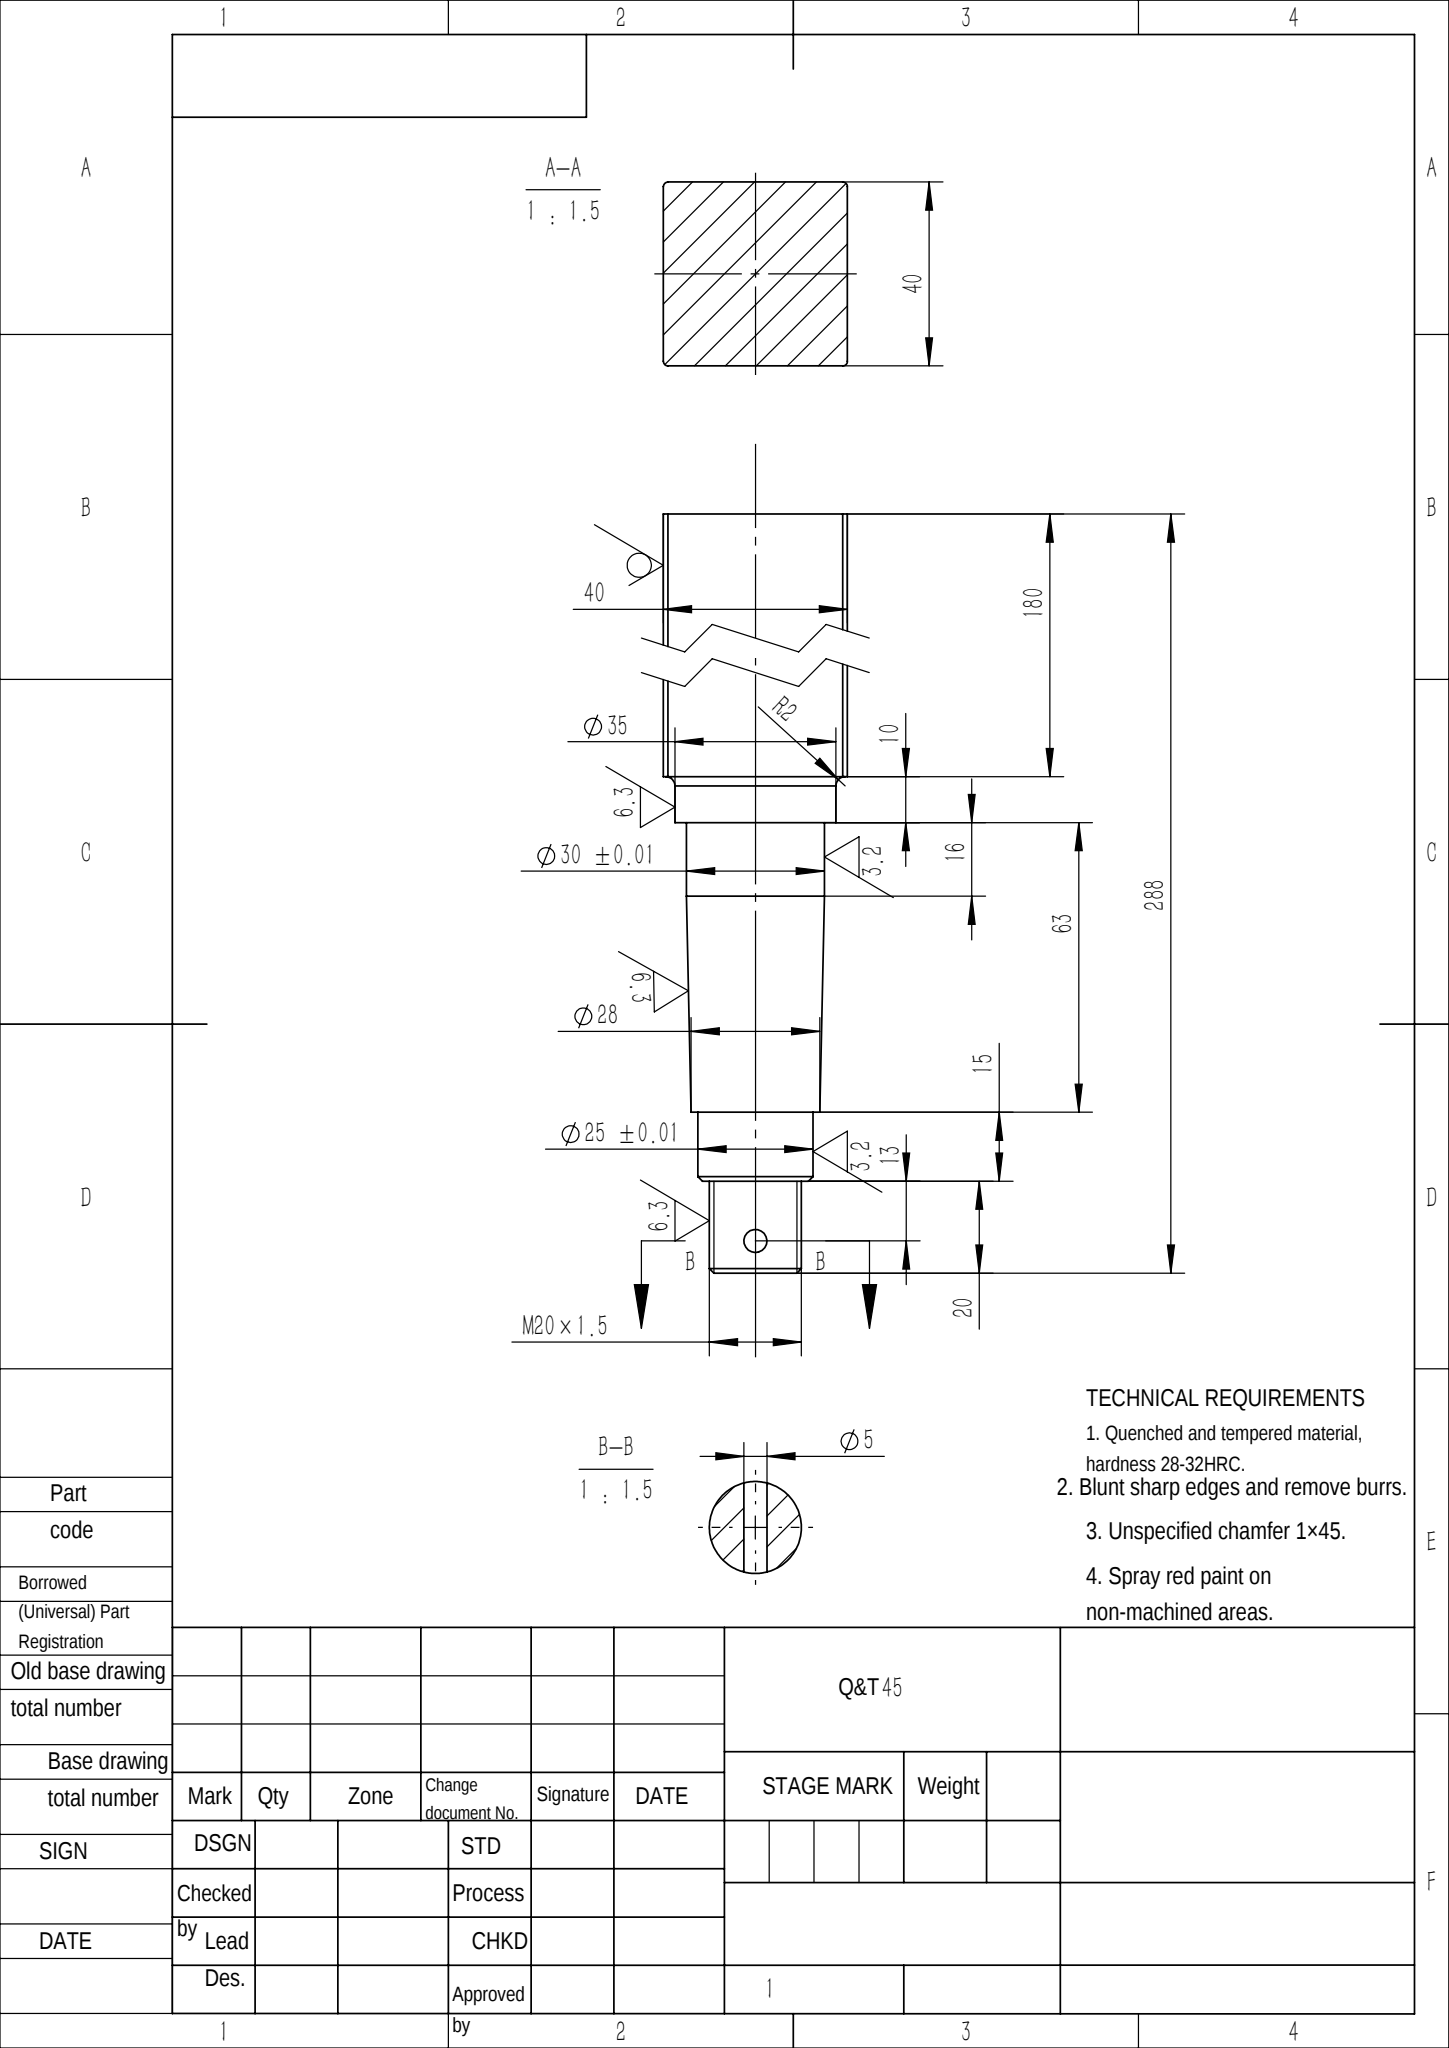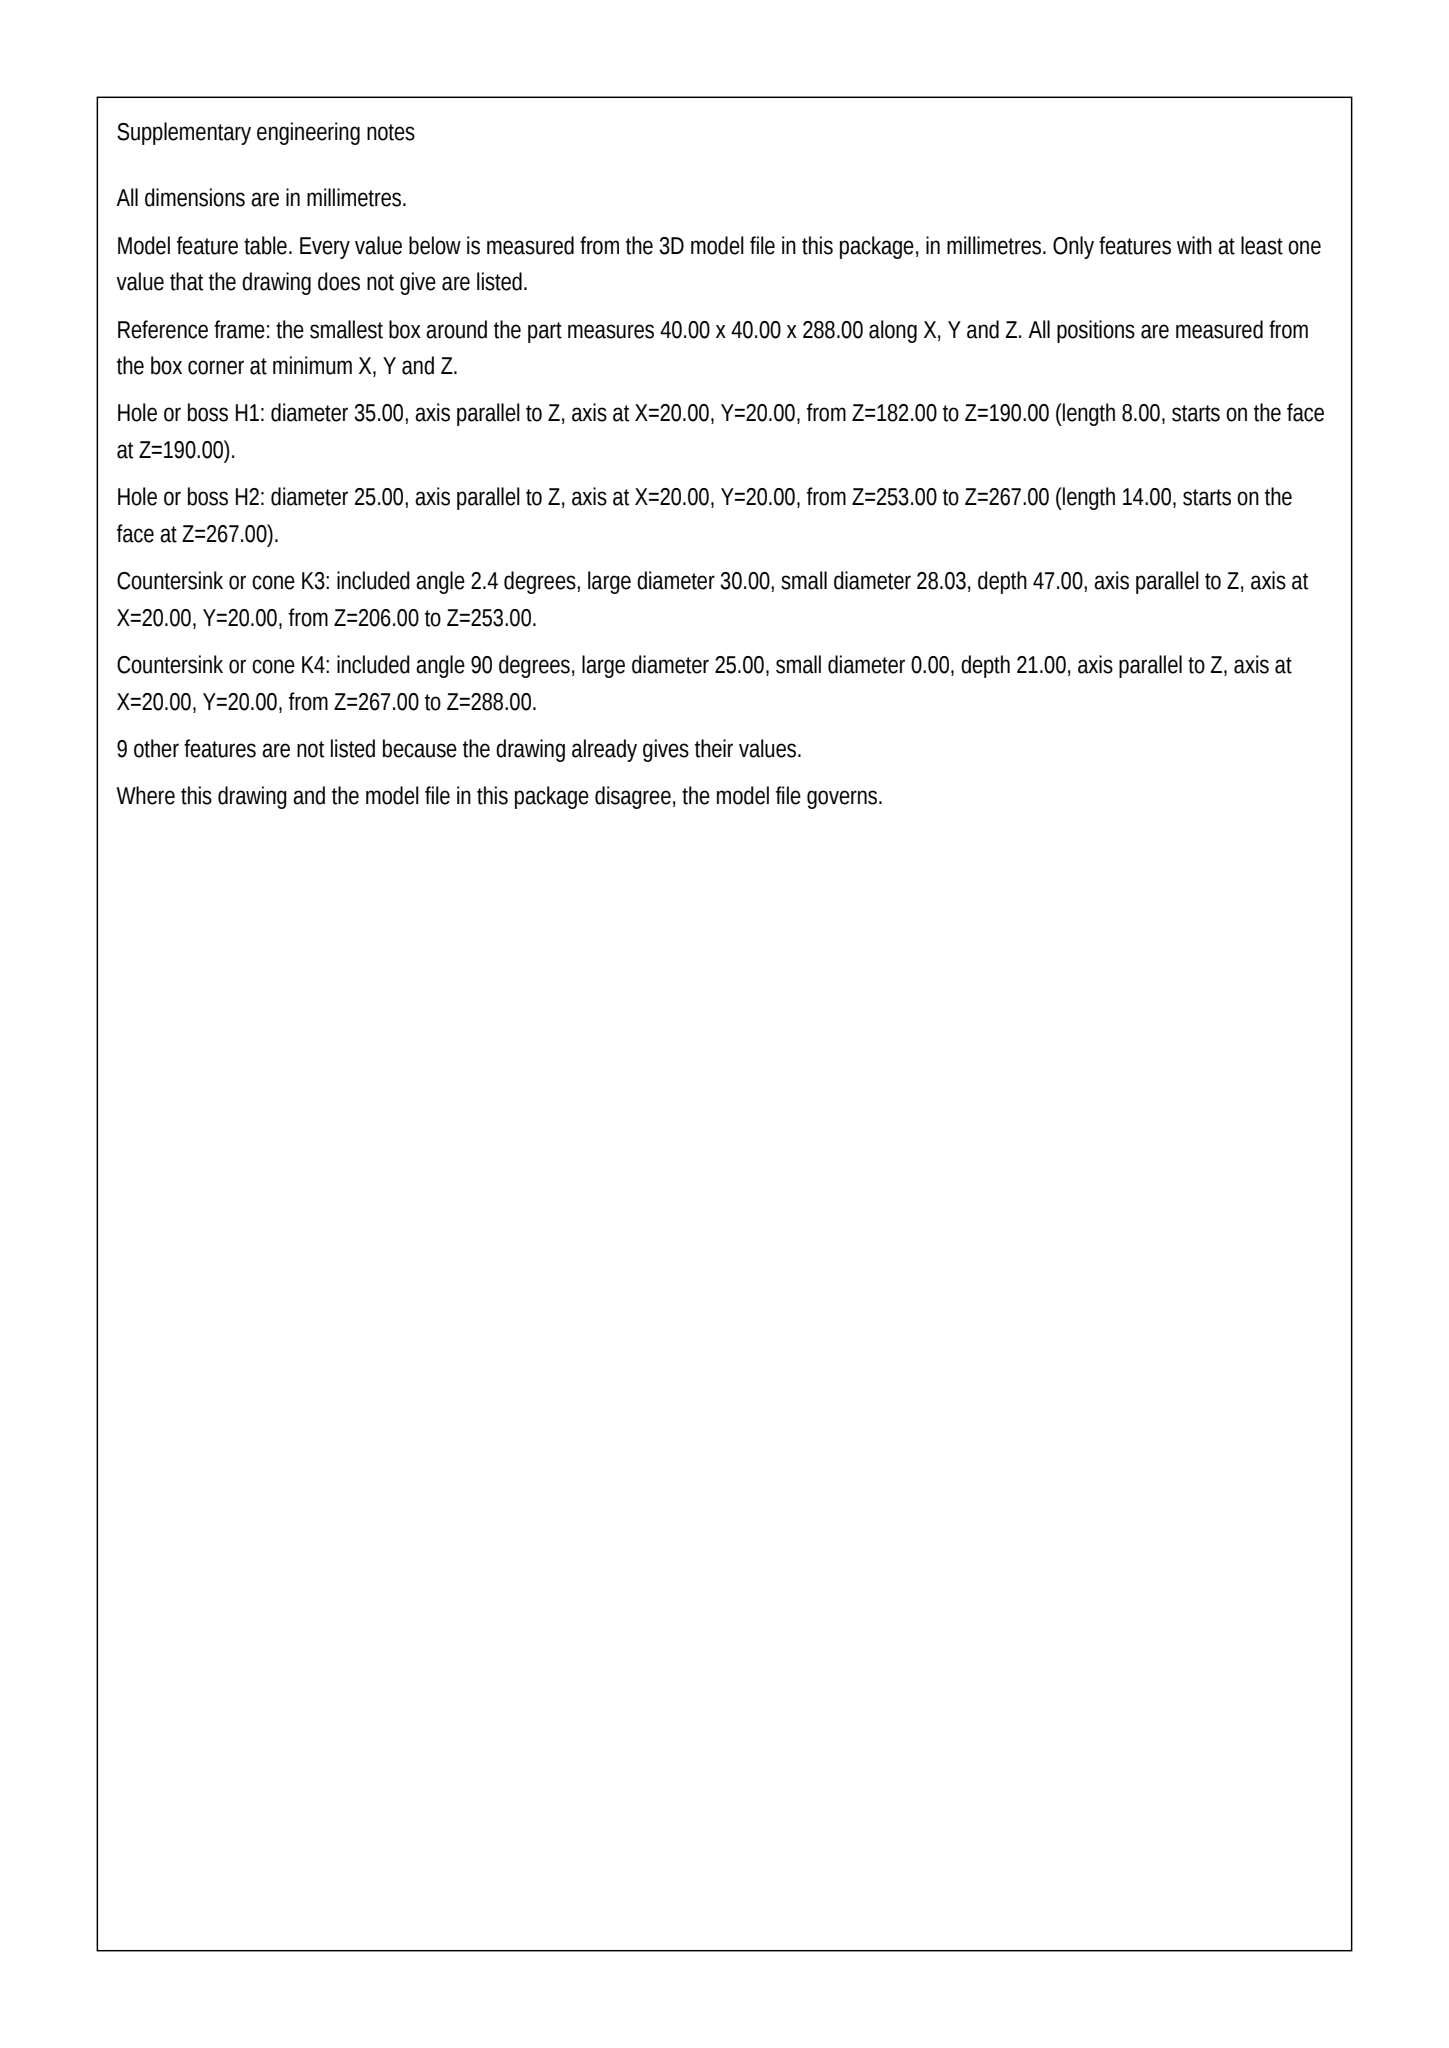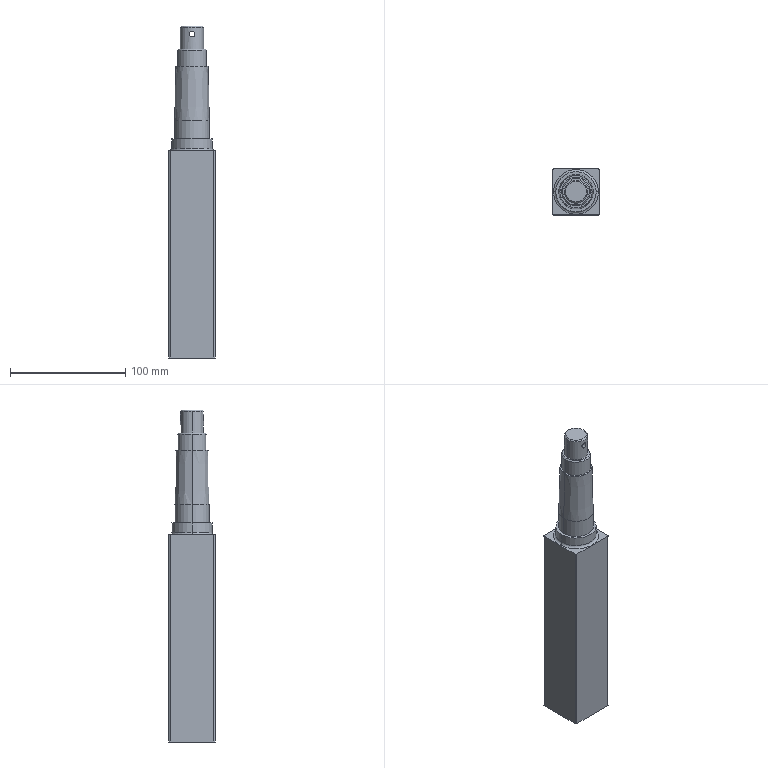Part | SolidWorks | mm | 1 solid | 32 faces | box 40 x 40 x 288 mm | volume 353118 mm3 | cylinder 14 | plane 10 | cone 6 | torus 2 | commonest cylinder face diameters 2 x4 5 x2 25 x2 20 x2 30 x2 35 x2